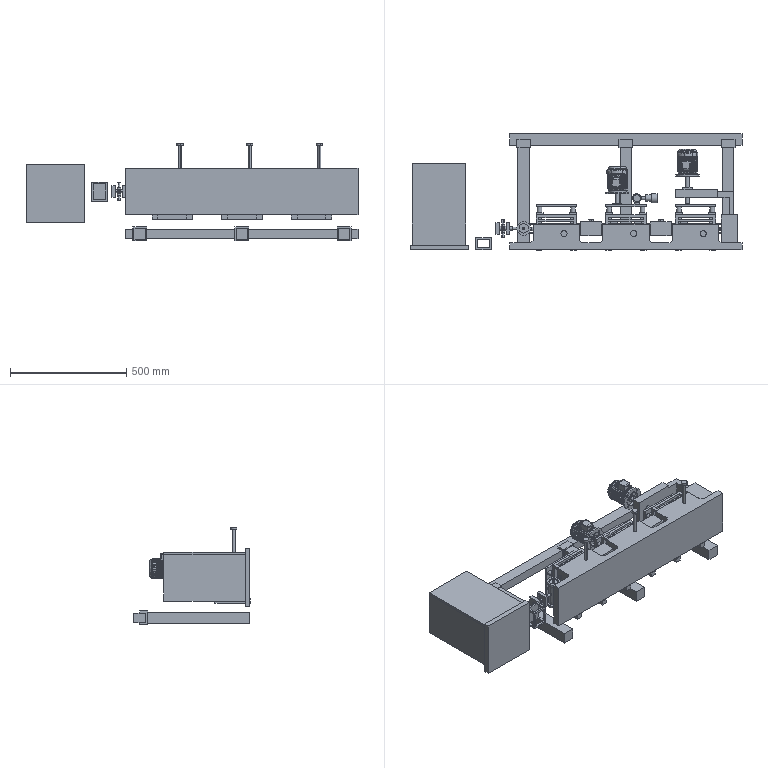Assembly | SolidWorks | mm | 69 component files | 73 solids | 3275 faces | box 1430 x 502 x 421.48 mm | volume 35353698 mm3 | plane 2538 | cylinder 515 | cone 206 | spline 12 | sphere 4 | commonest cylinder face diameters 1.5 x144 10 x66 6 x46 15 x40 20 x36 75 x22 12 x14 40 x12
Bill of materials:
Chassis | 1 |  | Rectangular block with a step along one long side: a lower ledge and a taller main section. The top face has a shallow raised or outlined rectangular panel with a row of four small short slot or bump features.
DriveStripAxis | 2 |  | Long, thin, solid straight cylindrical rod with flat ends.
DriveStripPlate | 4 |  | Thick circular disc with an annular recess in the top face and a small central hollow boss with a through-bore.
ElectricalBox | 1 |  | Rectangular box-like block with chamfered edges and a rectangular through-opening or pocket in one end face.
ElectricalCabinet | 1 |  | Open-top, thin-walled rectangular tray or box with one internal divider wall and a plate or flange at one end that sticks out past the body outline.
ElectricalCabinetPanel | 1 |  | Thin, flat rectangular plate with no visible holes or features.
InstrumentPanel | 1 |  | Compound body of cylinders: a short vertical cylinder with a circular groove or recess outline on its top face, a short side boss, and on the opposite side a thin rod leading to two coaxial stepped cylinders that grow in diameter.
LegSupport | 12 |  | Plain solid cylinder with flat ends and a length roughly comparable to its diameter.
Motor2 | 2 |  | Finned cylindrical housing with a circular mounting flange that has four holes, a protruding output shaft, a rectangular box on top, and a domed rear end cover. Its overall form resembles a flange-mounted electric motor.
MotorAxisHousing3 | 1 |  | Stepped solid cylindrical shaft or pin with two diameters: a longer large-diameter section and a shorter reduced-diameter section, joined by a shoulder.
MotorAxisHousingBase | 1 |  | Thick square plate or block with a large central circular through-hole, giving a square frame with a round opening.
MotorAxisHousingBase2 | 1 |  | Thin square plate with one central circular through-hole. Its shape resembles a square washer.
MotorMount | 1 |  | Rectangular open box frame (cage) made of square-section members along the edges, with large rectangular openings in the faces and at least one solid panel inside or on one face.
MotorShaftHousing | 1 |  | Long, straight, thin-walled circular tube with plain cut ends.
MotorShaftHousing2 | 1 |  | Short hollow cylindrical sleeve/tube with a moderately thick wall and plain ends.
MotorSupportPlate | 1 |  | Stepped L-shaped bracket: a flat rectangular plate with one small round through-hole, a perpendicular leg at one end, and stepped/narrowed tab sections.
OuterFlipShell | 1 |  | Two parallel thick square plates joined by a central fitting of intersecting hollow cylindrical tubes on three orthogonal axes; each plate has a central round through-hole.
OuterFlipStrip | 4 |  | Hollow cylindrical spacer/standoff with a thick wall and flat ends.
OuterRod | 1 |  | Long straight prismatic bar of rectangular, near-square cross-section with flat square-cut ends.
OuterRodSupport | 1 |  | Three identical, parallel, evenly spaced square-section bars, each ending in a fork/clip-shaped end with two thin prongs and a slightly wider head.
ProductionLineBase | 1 |  | Elongated rectangular rail/housing with a hollow rectangular end opening and three raised tabs along the top, each tab with small holes; there is a taller post at one end.
Shim | 6 |  | Simple solid rectangular block/bar with flat faces and no visible holes.
StripAxis | 3 |  | Headed pin: a straight cylindrical shank with a short, larger-diameter cylindrical head at one end and a plain opposite end.
SupportFastAxis | 2 |  | Very long, slender cylindrical rod with a small, slightly larger head at one end.
SupportFastAxisRing | 2 |  | Short hollow cylinder (annular ring/sleeve) with a concentric through bore; axial length is small relative to outer diameter.
SupportFrame | 3 |  | Bent/folded thin-wall bracket with a C/J-shaped side profile: a vertical web, a short top flange ending in a small downturned lip and containing a long slot, and a bottom that splits into two parallel prong-like arms separated by an open gap.
SupportPlate | 3 |  | Thin flat rectangular plate with no visible holes, cutouts, or edge features.
Track | 1 |  | Thin-walled hollow band or tube with an elongated obround (stadium-shaped) cross-section, open at both ends, long and narrow in plan with a modest height.
TrackDriveStrip | 2 |  | Solid cylindrical rod/spacer with a small concentric axial through hole; length is about 2.4 times the diameter.
TrackSupportBlock | 2 |  | Prismatic block with a constant I-shaped (double-T) cross-section extruded along its length, with one round hole in each flange region running along the extrusion direction.
Workpiece | 5 |  | Square plate (thick flange) with a single concentric cylindrical boss projecting from one face.
Mates:
1. coincident | ProductionLineBase-1 face at (500, 30, -100) dir (0, 0, -1) | SupportFrame-1 face at (-387, -2, -100) dir (0, 0, 1)
2. width | ProductionLineBase-1 face at (-400, 30, -315.407) dir (-1, 0, 0) | ProductionLineBase-1 face at (-200, 30, -315.407) dir (1, 0, 0) | SupportFrame-1 face at (-213, 150, 92) dir (1, 0, 0) | SupportFrame-1 face at (-387, 150, 92) dir (-1, 0, 0)
3. coincident | SupportFrame-1 face at (-387, 150, 92) dir (-1, 0, 0) | Shim-1 face at (-387, 160, -84) dir (-1, 0, 0)
4. distance | Shim-1 face at (-387, 160, 56) dir (0, 0, 1) | SupportFrame-1 face at (-387, 150, 92) dir (0, 0, 1)
5. coincident | SupportFrame-1 face at (-213, 150, 92) dir (1, 0, 0) | Shim-7 face at (-213, 160, -84) dir (1, 0, 0)
6. coincident | SupportFrame-1 face at (-81.735, 150, 12.053) dir (0, 1, 0) | Shim-7 face at (62.265, 150, 0.821) dir (0, -1, 0)
7. coincident | Shim-1 face at (-387, 160, 56) dir (0, 0, 1) | Shim-7 face at (-243, 160, 56) dir (0, 0, 1)
8. distance | LegSupport-1 plane at (-81.735, 160, -54) dir (0, 0, -1) | Shim-1 face at (-387, 160, -84) dir (0, 0, -1)
9. distance | Shim-1 face at (-387, 160, -84) dir (-1, 0, 0) | LegSupport-1 plane at (-372, 160, 0.821) dir (-1, 0, 0)
10. coincident | Shim-1 face at (-81.735, 160, 0.821) dir (0, 1, 0) | LegSupport-1 face at (-372, 160, -54) dir (0, -1, 0)
11. distance | LegSupport-17 plane at (-662.265, 160, 26) dir (0, 0, 1) | Shim-1 face at (-387, 160, 56) dir (0, 0, 1)
12. distance | Shim-1 face at (-387, 160, -84) dir (-1, 0, 0) | LegSupport-17 plane at (-372, 160, -28.821) dir (1, 0, 0)
13. coincident | Shim-1 face at (-81.735, 160, 0.821) dir (0, 1, 0) | LegSupport-17 face at (-372, 160, 26) dir (0, -1, 0)
14. coincident | Shim-7 face at (62.265, 160, 0.821) dir (0, 1, 0) | LegSupport-20 face at (-228, 160, -54) dir (0, -1, 0)
15. distance | LegSupport-20 plane at (62.265, 160, -54) dir (0, 0, -1) | Shim-7 face at (-243, 160, -84) dir (0, 0, -1)
16. distance | Shim-7 face at (-243, 160, -84) dir (-1, 0, 0) | LegSupport-20 plane at (-228, 160, 0.821) dir (-1, 0, 0)
17. distance | LegSupport-23 plane at (62.265, 160, 26) dir (0, 0, -1) | Shim-7 face at (-243, 160, 56) dir (0, 0, 1)
18. distance | Shim-7 face at (-243, 160, -84) dir (-1, 0, 0) | LegSupport-23 plane at (-228, 160, 80.821) dir (-1, 0, 0)
19. coincident | Shim-7 face at (62.265, 160, 0.821) dir (0, 1, 0) | LegSupport-23 face at (-228, 160, 26) dir (0, -1, 0)
20. coincident | Shim-1 face at (-387, 160, -84) dir (-1, 0, 0) | SupportPlate-2 face at (-387, 195, 56) dir (-1, 0, 0)
21. coincident | LegSupport-1 face at (-372, 185, -54) dir (0, 1, 0) | SupportPlate-2 face at (-81.735, 185, 0.821) dir (0, -1, 0)
22. coincident | Shim-7 face at (-243, 160, 56) dir (0, 0, 1) | SupportPlate-2 face at (-213, 195, 56) dir (0, 0, 1)
23. distance | ProductionLineBase-1 face at (-100, 30, -315.407) dir (-1, 0, 0) | TrackSupportBlock-2 face at (-105, -1.434, 0) dir (1, 0, 0)
24. coincident | ProductionLineBase-1 face at (500, 60, -50) dir (0, 1, 0) | TrackSupportBlock-2 face at (-195, 60, 50) dir (0, -1, 0)
25. coincident | TrackSupportBlock-2 face at (-195, 120, 50) dir (0, 0, -1) | Track-1 face at (-440, 92, 50) dir (0, 0, 1)
26. distance | Track-1 edge at (-440, 112, 50) dir (0, 0, -1) | ProductionLineBase-1 face at (-400, 30, -315.407) dir (-1, 0, 0)
27. concentric | Track-1 face at (-440, 92, 50) dir (0, 0, -1) r 17 | TrackDriveStrip-2 face at (-440, 92, -50) dir (0, 0, 1) r 17
28. concentric | TrackDriveStrip-2 face at (-440, 92, -50) dir (0, 0, 1) r 3 | DriveStripAxis-2 face at (-440, 92, -65) dir (0, 0, 1) r 3
29. distance | DriveStripAxis-2 face at (-440, 92, -65) dir (0, 0, -1) | TrackDriveStrip-2 face at (-440, 92, -50) dir (0, 0, -1)
30. coincident | Track-1 face at (-440, 92, -50) dir (0, 0, -1) | TrackDriveStrip-2 face at (-440, 92, -50) dir (0, 0, -1)
31. concentric | DriveStripAxis-2 face at (-440, 92, -65) dir (0, 0, 1) r 3 | DriveStripPlate-1 face at (-440, 92, 55) dir (0, 0, -1) r 3
32. coincident | TrackDriveStrip-2 face at (-440, 92, 50) dir (0, 0, 1) | DriveStripPlate-1 face at (-440, 92, 50) dir (0, 0, -1)
33. coincident | ProductionLineBase-1 face at (500, 160, 50) dir (0, 0, -1) | TrackSupportBlock-2 face at (-195, 120, 50) dir (0, 0, -1)
34. concentric | ProductionLineBase-1 face at (-500, 90, 65) dir (1, 0, 0) r 5 | SupportFastAxis-2 face at (406, 90, 65) dir (-1, 0, 0) r 5
35. coincident | ProductionLineBase-1 face at (-400, 30, -315.407) dir (-1, 0, 0) | SupportFastAxis-2 face at (-400, 90, 65) dir (1, 0, 0)
36. concentric | SupportFastAxis-2 face at (406, 90, 65) dir (-1, 0, 0) r 5 | SupportFastAxisRing-2 face at (405, 90, 65) dir (-1, 0, 0) r 5
37. coincident | ProductionLineBase-1 face at (400, 30, -315.407) dir (1, 0, 0) | SupportFastAxisRing-2 face at (400, 90, 65) dir (-1, 0, 0)
38. distance | ElectricalCabinet-2 face at (-680, 0, 115) dir (1, 0, 0) | ProductionLineBase-1 face at (-500, 30, 100) dir (-1, 0, 0)
39. distance | ElectricalCabinet-2 face at (-930, 0, 115) dir (0, 0, 1) | ProductionLineBase-1 face at (500, 30, 100) dir (0, 0, 1)
40. coincident | ProductionLineBase-1 face at (0, 0, 0) dir (0, -1, 0) | ElectricalCabinet-2 face at (-690, 0, -10) dir (0, -1, 0)
41. coincident | ProductionLineBase-1 face at (-400, 110, -315.407) dir (0, 1, 0) | SupportFrame-1 face at (-81.735, 110, 12.053) dir (0, -1, 0)
42. coincident | SupportFrame-1 face at (-81.735, 150, 12.053) dir (0, 1, 0) | Shim-1 face at (-81.735, 150, 0.821) dir (0, -1, 0)
43. coincident | ElectricalCabinet-2 face at (-920, 370, -110) dir (0, 1, 0) | ElectricalCabinetPanel-2 face at (-920, 370, 100) dir (0, 1, 0)
44. coincident | ElectricalCabinet-2 face at (-920, 20, -10) dir (-1, 0, 0) | ElectricalCabinetPanel-2 face at (-920, 370, 100) dir (-1, 0, 0)
45. coincident | ElectricalCabinet-2 face at (-920, 20, 90) dir (0, 0, 1) | ElectricalCabinetPanel-2 face at (-690, 20, 90) dir (0, 0, -1)
46. coincident | ElectricalCabinet-2 face at (-910, 260, 80) dir (0, 1, 0) | Chassis-2 face at (-695, 260, -10) dir (0, -1, 0)
47. coincident | ElectricalCabinet-2 face at (-910, 20, -10) dir (1, 0, 0) | Chassis-2 face at (-910, 350, -100) dir (-1, 0, 0)
48. coincident | ElectricalCabinet-2 face at (-920, 20, -100) dir (0, 0, 1) | Chassis-2 face at (-910, 350, -100) dir (0, 0, -1)
49. coincident | ElectricalCabinet-2 face at (-730, 155, -50) dir (0, 1, 0) | ElectricalBox-2 face at (-690, 155, -10) dir (0, -1, 0)
50. coincident | ElectricalCabinet-2 face at (-920, 20, -100) dir (0, 0, 1) | ElectricalBox-2 face at (-735, 205, -100) dir (0, 0, -1)
51. coincident | ElectricalCabinet-2 face at (-810, 155, -50) dir (-1, 0, 0) | ElectricalBox-2 face at (-810, 205, -100) dir (-1, 0, 0)
52. width | OuterRod-1 face at (-500, 500, -162.763) dir (-1, 0, 0) | OuterRod-1 face at (500, 500, -162.763) dir (1, 0, 0) | OuterRodSupport-1 face at (-465, 440, -207.763) dir (-1, 0, 0) | OuterRodSupport-1 face at (465, 440, -207.763) dir (1, 0, 0)
53. coincident | SupportPlate-4 face at (518.265, 195, 0.821) dir (0, 1, 0) | MotorAxisHousingBase-2 face at (528.265, 195, -9.179) dir (0, -1, 0)
54. concentric | MotorAxisHousingBase-2 face at (265, 200, 30) dir (0, -1, 0) r 7.5 | MotorShaftHousing-2 face at (265, 173.787, 30) dir (0, 1, 0) r 7.5
55. coincident | SupportPlate-3 face at (218.265, 195, 0.821) dir (0, 1, 0) | MotorAxisHousingBase2-2 face at (259.282, 195, -14) dir (0, -1, 0)
56. distance | MotorAxisHousingBase2-2 face at (-57, 200, 26) dir (-1, 0, 0) | SupportPlate-3 face at (-87, 195, 56) dir (-1, 0, 0)
57. distance | SupportPlate-3 face at (87, 195, 56) dir (0, 0, 1) | MotorAxisHousingBase2-2 face at (-17, 200, 26) dir (0, 0, 1)
58. concentric | MotorAxisHousingBase2-2 face at (-37, 200, 6) dir (0, -1, 0) r 7.5 | MotorShaftHousing2-2 face at (-37, 267.963, 6) dir (0, -1, 0) r 7.5
59. coincident | SupportPlate-3 face at (218.265, 195, 0.821) dir (0, 1, 0) | MotorShaftHousing2-2 face at (-37, 195, 6) dir (0, -1, 0)
60. concentric | MotorShaftHousing2-2 face at (-37, 267.963, 6) dir (0, -1, 0) r 4.75 | Motor2-1 face at (-37, 222.25, 6) dir (0, 1, 0) r 4.75
61. coincident | MotorShaftHousing2-2 face at (-29.418, 246.75, 9.252) dir (0, 1, 0) | Motor2-1 face at (-37, 246.75, 6) dir (0, -1, 0)
62. concentric | MotorShaftHousing-2 edge at (265, 321.75, 30) dir (0, 1, 0) r 4.75 | Motor2-2 face at (265, 297.25, 30) dir (0, 1, 0) r 4.75
63. coincident | MotorShaftHousing-2 face at (270.632, 321.75, 36.028) dir (0, 1, 0) | Motor2-2 face at (265, 321.75, 30) dir (0, -1, 0)
64. coincident | ProductionLineBase-1 face at (500, 30, 100) dir (0, 0, 1) | assembly face at (-400, 28, 100) dir (0, 0, -1)
65. parallel | ProductionLineBase-1 face at (0, 0, 0) dir (0, -1, 0) | assembly face at (-400, 28, 105.6) dir (0, -1, 0)
66. coincident | ProductionLineBase-1 face at (-400, 30, -315.407) dir (-1, 0, 0) | assembly face at (-400, 94, 100) dir (-1, 0, 0)
67. coincident | ProductionLineBase-1 face at (-400, 110, -315.407) dir (0, 1, 0) | assembly face at (-400, 110, 105.6) dir (0, 1, 0)
68. concentric | assembly face at (-366, 69, 140) dir (-1, 0, 0) r 5.6 | assembly face at (-268.908, 69, 140) dir (-1, 0, 0) r 6
69. coincident | assembly face at (-291.2, 67.4, 146.8) dir (0, -1, 0) | assembly face at (-297.109, 67.4, 146.8) dir (0, 1, 0)
70. coincident | assembly face at (-288.8, 69, 144.76) dir (1, 0, 0) | assembly face at (-288.8, 69, 140) dir (1, 0, 0)
71. concentric | StripAxis-1 face at (-266.709, 69.045, 55) dir (0, 0, 1) r 6 | assembly face at (-266.709, 69.045, 142.519) dir (0, 0, 1) r 6
72. distance | assembly face at (-266.709, 69.045, 170.72) dir (0, 0, 1) | StripAxis-1 face at (-266.709, 69.045, 198.72) dir (0, 0, -1)
73. concentric | StripAxis-1 face at (-266.709, 69.045, 198.72) dir (0, 0, 1) r 13 | assembly face at (-266.709, 69.045, 198.72) dir (0, 0, 1) r 13
74. coincident | StripAxis-1 face at (-266.709, 69.045, 208.72) dir (0, 0, 1) | assembly face at (-367.326, 69.045, 208.72) dir (0, 0, 1)
75. parallel | assembly face at (-339.4, 89.12, 204.784) dir (0, 1, 0) | assembly face at (-367.326, 84.045, 198.72) dir (0, 1, 0)
76. distance | assembly edge at (-266.709, 84.045, 198.72) dir (0, 0, 1) | assembly edge at (-339.4, 90.76, 204.784) dir (0, 0, 1)
77. coincident | assembly face at (-339.4, 52.816, 208.72) dir (0, 0, 1) | assembly face at (-367.326, 69.045, 208.72) dir (0, 0, 1)
78. distance | assembly face at (-339.4, 90.76, 208.72) dir (0, 1, 0) | assembly face at (-367.326, 84.045, 198.72) dir (0, 1, 0)
79. concentric | assembly face at (-66, 69, 140) dir (-1, 0, 0) r 5.6 | assembly face at (31.092, 69, 140) dir (-1, 0, 0) r 6
80. coincident | assembly face at (8.8, 67.4, 146.8) dir (0, -1, 0) | assembly face at (2.891, 67.4, 146.8) dir (0, 1, 0)
81. coincident | assembly face at (11.2, 69, 144.76) dir (1, 0, 0) | assembly face at (11.2, 69, 140) dir (1, 0, 0)
82. concentric | StripAxis-7 face at (33.291, 69.045, 55) dir (0, 0, 1) r 6 | assembly face at (33.291, 69.045, 142.519) dir (0, 0, 1) r 6
83. distance | assembly face at (33.291, 69.045, 170.72) dir (0, 0, 1) | StripAxis-7 face at (33.291, 69.045, 198.72) dir (0, 0, -1)
84. concentric | StripAxis-7 face at (33.291, 69.045, 198.72) dir (0, 0, 1) r 13 | assembly face at (33.291, 69.045, 198.72) dir (0, 0, 1) r 13
85. coincident | StripAxis-7 face at (33.291, 69.045, 208.72) dir (0, 0, 1) | assembly face at (-67.326, 69.045, 208.72) dir (0, 0, 1)
86. parallel | assembly face at (-39.4, 89.12, 204.784) dir (0, 1, 0) | assembly face at (-67.326, 84.045, 198.72) dir (0, 1, 0)
87. distance | assembly edge at (33.291, 84.045, 198.72) dir (0, 0, 1) | assembly edge at (-39.4, 90.76, 204.784) dir (0, 0, 1)
88. coincident | assembly face at (-39.4, 52.816, 208.72) dir (0, 0, 1) | assembly face at (-67.326, 69.045, 208.72) dir (0, 0, 1)
89. distance | assembly face at (-39.4, 90.76, 208.72) dir (0, 1, 0) | assembly face at (-67.326, 84.045, 198.72) dir (0, 1, 0)
90. coincident | ProductionLineBase-1 face at (500, 30, 100) dir (0, 0, 1) | assembly face at (-100, 28, 100) dir (0, 0, -1)
91. coincident | ProductionLineBase-1 face at (-100, 30, -315.407) dir (-1, 0, 0) | assembly face at (-100, 94, 100) dir (-1, 0, 0)
92. coincident | ProductionLineBase-1 face at (-100, 110, -315.407) dir (0, 1, 0) | assembly face at (-100, 110, 105.6) dir (0, 1, 0)
93. concentric | assembly face at (234, 69, 140) dir (-1, 0, 0) r 5.6 | assembly face at (331.092, 69, 140) dir (-1, 0, 0) r 6
94. coincident | assembly face at (308.8, 67.4, 146.8) dir (0, -1, 0) | assembly face at (302.891, 67.4, 146.8) dir (0, 1, 0)
95. coincident | assembly face at (311.2, 69, 144.76) dir (1, 0, 0) | assembly face at (311.2, 69, 140) dir (1, 0, 0)
96. concentric | StripAxis-9 face at (333.291, 69.045, 55) dir (0, 0, 1) r 6 | assembly face at (333.291, 69.045, 142.519) dir (0, 0, 1) r 6
97. distance | assembly face at (333.291, 69.045, 170.72) dir (0, 0, 1) | StripAxis-9 face at (333.291, 69.045, 198.72) dir (0, 0, -1)
98. concentric | StripAxis-9 face at (333.291, 69.045, 198.72) dir (0, 0, 1) r 13 | assembly face at (333.291, 69.045, 198.72) dir (0, 0, 1) r 13
99. coincident | StripAxis-9 face at (333.291, 69.045, 208.72) dir (0, 0, 1) | assembly face at (232.674, 69.045, 208.72) dir (0, 0, 1)
100. parallel | assembly face at (260.6, 89.12, 204.784) dir (0, 1, 0) | assembly face at (232.674, 84.045, 198.72) dir (0, 1, 0)
101. distance | assembly edge at (333.291, 84.045, 198.72) dir (0, 0, 1) | assembly edge at (260.6, 90.76, 204.784) dir (0, 0, 1)
102. coincident | assembly face at (260.6, 52.816, 208.72) dir (0, 0, 1) | assembly face at (232.674, 69.045, 208.72) dir (0, 0, 1)
103. distance | assembly face at (260.6, 90.76, 208.72) dir (0, 1, 0) | assembly face at (232.674, 84.045, 198.72) dir (0, 1, 0)
104. coincident | ProductionLineBase-1 face at (500, 30, 100) dir (0, 0, 1) | assembly face at (200, 28, 100) dir (0, 0, -1)
105. coincident | ProductionLineBase-1 face at (200, 30, -315.407) dir (-1, 0, 0) | assembly face at (200, 94, 100) dir (-1, 0, 0)
106. coincident | ProductionLineBase-1 face at (200, 110, -315.407) dir (0, 1, 0) | assembly face at (200, 110, 105.6) dir (0, 1, 0)
107. parallel | ProductionLineBase-1 face at (0, 30, 0) dir (0, 1, 0) | assembly face at (-647.2, 52, 41) dir (0, -1, 0)
108. concentric | assembly face at (-613.2, 92, 0) dir (-1, 0, 0) r 5.6 | MotorAxisHousing3-1 face at (-490, 92, 0) dir (-1, 0, 0) r 5.6
109. coincident | assembly face at (-560, 99, 0) dir (1, 0, 0) | MotorAxisHousing3-1 face at (-560, 92, 0) dir (-1, 0, 0)
110. tangent | OuterFlipShell-1 face at (-515, 92, 0) dir (-1, 0, 0) r 8.5 | OuterFlipStrip-2 face at (-530, 92, 8.5) dir (0, 0, -1)
111. concentric | OuterFlipShell-1 face at (-530, 92, 18.5) dir (0, 0, -1) r 5 | OuterFlipStrip-2 face at (-530, 92, 38.5) dir (0, 0, -1) r 5
112. tangent | OuterFlipShell-1 face at (-515, 92, 0) dir (-1, 0, 0) r 8.5 | OuterFlipStrip-3 face at (-530, 100.5, 0) dir (0, -1, 0)
113. concentric | OuterFlipShell-1 face at (-530, 110.5, 0) dir (0, -1, 0) r 5 | OuterFlipStrip-3 face at (-530, 130.5, 0) dir (0, -1, 0) r 5
114. tangent | OuterFlipShell-1 face at (-515, 92, 0) dir (-1, 0, 0) r 8.5 | OuterFlipStrip-5 face at (-530, 83.5, 0) dir (0, 1, 0)
115. concentric | OuterFlipShell-1 face at (-530, 73.5, 0) dir (0, 1, 0) r 5 | OuterFlipStrip-5 face at (-530, 53.5, 0) dir (0, 1, 0) r 5
116. tangent | OuterFlipShell-1 face at (-515, 92, 0) dir (-1, 0, 0) r 8.5 | OuterFlipStrip-7 face at (-530, 92, -8.5) dir (0, 0, 1)
117. concentric | OuterFlipShell-1 face at (-530, 92, -18.5) dir (0, 0, 1) r 5 | OuterFlipStrip-7 face at (-530, 92, -38.5) dir (0, 0, 1) r 5
118. width | TrackSupportBlock-2 face at (-195, 120, 80) dir (0, 0, 1) | TrackSupportBlock-2 face at (-105, -1.434, -80) dir (0, 0, -1) | Workpiece-2 face at (-164.926, 122, 15) dir (0, 0, 1) | Workpiece-2 face at (-164.926, 122, -15) dir (0, 0, -1)
119. distance | Track-1 face at (-440, 72, 50) dir (0, -1, 0) | ProductionLineBase-1 face at (0, 30, 0) dir (0, 1, 0)